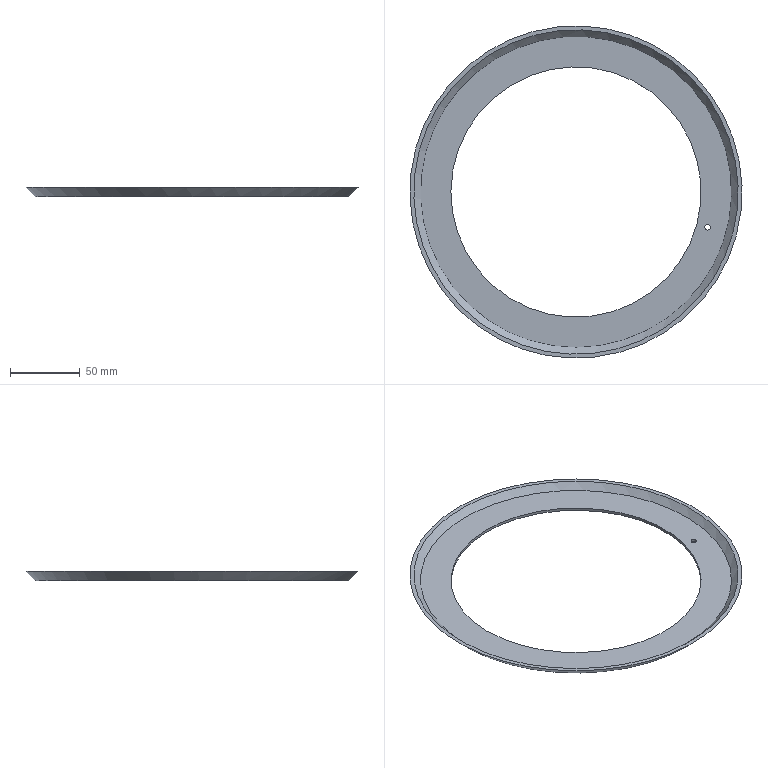Component | NX | OILTHROWRING_2 | 1 solid | 7 faces | box 239 x 239 x 6.75 mm | volume 40152 mm3 | plane 3 | cone 2 | cylinder 2 | commonest cylinder face diameters 4 x1 180 x1
STEP:
#1=CARTESIAN_POINT('',(0.,0.,0.));
#2=DIRECTION('',(0.,0.,1.));
#3=DIRECTION('',(1.,0.,0.));
#4=AXIS2_PLACEMENT_3D('',#1,#2,#3);
#5=CARTESIAN_POINT('',(-108.904,29.181,24.));
#6=VERTEX_POINT('',#5);
#7=CARTESIAN_POINT('',(-0.,0.,24.));
#8=DIRECTION('',(0.,-0.,-1.));
#9=DIRECTION('',(-0.9659,0.2588,-0.));
#10=AXIS2_PLACEMENT_3D('',#7,#8,#9);
#11=CIRCLE('',#10,112.745);
#12=CARTESIAN_POINT('',(108.904,-29.181,24.));
#13=DIRECTION('',(-0.,0.,1.));
#14=DIRECTION('',(0.9659,-0.2588,0.));
#15=AXIS2_PLACEMENT_3D('',#12,#13,#14);
#16=PLANE('',#15);
#17=CARTESIAN_POINT('',(-225.491,0.));
#18=CARTESIAN_POINT('',(-225.491,195.281));
#19=CARTESIAN_POINT('',(-56.373,97.64));
#20=CARTESIAN_POINT('',(112.745,0.));
#21=CARTESIAN_POINT('',(-56.373,-97.64));
#22=CARTESIAN_POINT('',(-225.491,-195.281));
#23=CARTESIAN_POINT('',(-225.491,0.));
#24=(BOUNDED_CURVE()B_SPLINE_CURVE(2,(#17,#18,#19,#20,#21,#22,#23),.UNSPECIFIED.,.T.,.F.)B_SPLINE_CURVE_WITH_KNOTS((1,2,2,2,2,1),(-2.094,0.,2.094,4.189,6.283,8.378),.UNSPECIFIED.)CURVE()GEOMETRIC_REPRESENTATION_ITEM()RATIONAL_B_SPLINE_CURVE((1.,0.5,1.,0.5,1.,0.5,1.))REPRESENTATION_ITEM(''));
#25=(GEOMETRIC_REPRESENTATION_CONTEXT(2)PARAMETRIC_REPRESENTATION_CONTEXT()REPRESENTATION_CONTEXT('',''));
#26=DEFINITIONAL_REPRESENTATION('',(#24),#25);
#27=PCURVE('',#16,#26);
#28=CARTESIAN_POINT('',(-0.,0.,30.755));
#29=DIRECTION('',(-0.,0.,1.));
#30=DIRECTION('',(0.9659,-0.2588,0.));
#31=AXIS2_PLACEMENT_3D('',#28,#29,#30);
#32=CONICAL_SURFACE('',#31,119.5,0.7854);
#33=CARTESIAN_POINT('',(9.425,-6.755));
#34=DIRECTION('',(-1.,0.));
#35=VECTOR('',#34,1.);
#36=LINE('',#33,#35);
#37=(GEOMETRIC_REPRESENTATION_CONTEXT(2)PARAMETRIC_REPRESENTATION_CONTEXT()REPRESENTATION_CONTEXT('',''));
#38=DEFINITIONAL_REPRESENTATION('',(#36),#37);
#39=PCURVE('',#32,#38);
#40=SURFACE_CURVE('',#11,(#27,#39),.PCURVE_S1.);
#41=EDGE_CURVE('',#6,#6,#40,.T.);
#42=ORIENTED_EDGE('',*,*,#41,.T.);
#43=EDGE_LOOP('',(#42));
#44=FACE_BOUND('',#43,.T.);
#45=CARTESIAN_POINT('',(96.593,-25.882,24.));
#46=VERTEX_POINT('',#45);
#47=CARTESIAN_POINT('',(94.661,-25.364,24.));
#48=DIRECTION('',(-0.,0.,1.));
#49=DIRECTION('',(0.9659,-0.2588,0.));
#50=AXIS2_PLACEMENT_3D('',#47,#48,#49);
#51=CIRCLE('',#50,2.);
#52=CARTESIAN_POINT('',(-14.745,0.));
#53=DIRECTION('',(1.,0.));
#54=AXIS2_PLACEMENT_2D('',#52,#53);
#55=CIRCLE('',#54,2.);
#56=(GEOMETRIC_REPRESENTATION_CONTEXT(2)PARAMETRIC_REPRESENTATION_CONTEXT()REPRESENTATION_CONTEXT('',''));
#57=DEFINITIONAL_REPRESENTATION('',(#55),#56);
#58=PCURVE('',#16,#57);
#59=CARTESIAN_POINT('',(94.661,-25.364,24.));
#60=DIRECTION('',(-0.,0.,1.));
#61=DIRECTION('',(0.9659,-0.2588,0.));
#62=AXIS2_PLACEMENT_3D('',#59,#60,#61);
#63=CYLINDRICAL_SURFACE('',#62,2.);
#64=CARTESIAN_POINT('',(0.,0.));
#65=DIRECTION('',(1.,0.));
#66=VECTOR('',#65,1.);
#67=LINE('',#64,#66);
#68=(GEOMETRIC_REPRESENTATION_CONTEXT(2)PARAMETRIC_REPRESENTATION_CONTEXT()REPRESENTATION_CONTEXT('',''));
#69=DEFINITIONAL_REPRESENTATION('',(#67),#68);
#70=PCURVE('',#63,#69);
#71=SURFACE_CURVE('',#51,(#58,#70),.PCURVE_S1.);
#72=EDGE_CURVE('',#46,#46,#71,.T.);
#73=ORIENTED_EDGE('',*,*,#72,.T.);
#74=EDGE_LOOP('',(#73));
#75=FACE_BOUND('',#74,.T.);
#76=CARTESIAN_POINT('',(86.933,-23.294,24.));
#77=VERTEX_POINT('',#76);
#78=CARTESIAN_POINT('',(-0.,0.,24.));
#79=DIRECTION('',(0.,-0.,-1.));
#80=DIRECTION('',(0.9659,-0.2588,0.));
#81=AXIS2_PLACEMENT_3D('',#78,#79,#80);
#82=CIRCLE('',#81,90.);
#83=CARTESIAN_POINT('',(-22.745,0.));
#84=CARTESIAN_POINT('',(-22.745,-155.885));
#85=CARTESIAN_POINT('',(-157.745,-77.942));
#86=CARTESIAN_POINT('',(-292.745,0.));
#87=CARTESIAN_POINT('',(-157.745,77.942));
#88=CARTESIAN_POINT('',(-22.745,155.885));
#89=CARTESIAN_POINT('',(-22.745,0.));
#90=(BOUNDED_CURVE()B_SPLINE_CURVE(2,(#83,#84,#85,#86,#87,#88,#89),.UNSPECIFIED.,.T.,.F.)B_SPLINE_CURVE_WITH_KNOTS((1,2,2,2,2,1),(-2.094,0.,2.094,4.189,6.283,8.378),.UNSPECIFIED.)CURVE()GEOMETRIC_REPRESENTATION_ITEM()RATIONAL_B_SPLINE_CURVE((1.,0.5,1.,0.5,1.,0.5,1.))REPRESENTATION_ITEM(''));
#91=(GEOMETRIC_REPRESENTATION_CONTEXT(2)PARAMETRIC_REPRESENTATION_CONTEXT()REPRESENTATION_CONTEXT('',''));
#92=DEFINITIONAL_REPRESENTATION('',(#90),#91);
#93=PCURVE('',#16,#92);
#94=CARTESIAN_POINT('',(-0.,0.,26.));
#95=DIRECTION('',(0.,-0.,-1.));
#96=DIRECTION('',(-0.9659,0.2588,-0.));
#97=AXIS2_PLACEMENT_3D('',#94,#95,#96);
#98=CYLINDRICAL_SURFACE('',#97,90.);
#99=CARTESIAN_POINT('',(3.142,2.));
#100=DIRECTION('',(1.,0.));
#101=VECTOR('',#100,1.);
#102=LINE('',#99,#101);
#103=(GEOMETRIC_REPRESENTATION_CONTEXT(2)PARAMETRIC_REPRESENTATION_CONTEXT()REPRESENTATION_CONTEXT('',''));
#104=DEFINITIONAL_REPRESENTATION('',(#102),#103);
#105=PCURVE('',#98,#104);
#106=SURFACE_CURVE('',#82,(#93,#105),.PCURVE_S1.);
#107=EDGE_CURVE('',#77,#77,#106,.T.);
#108=ORIENTED_EDGE('',*,*,#107,.F.);
#109=EDGE_LOOP('',(#108));
#110=FACE_BOUND('',#109,.T.);
#111=ADVANCED_FACE('',(#44,#75,#110),#16,.F.);
#112=CARTESIAN_POINT('',(-112.696,30.197,30.755));
#113=VERTEX_POINT('',#112);
#114=CARTESIAN_POINT('',(-0.,0.,30.755));
#115=DIRECTION('',(0.,-0.,-1.));
#116=DIRECTION('',(-0.9659,0.2588,-0.));
#117=AXIS2_PLACEMENT_3D('',#114,#115,#116);
#118=CIRCLE('',#117,116.672);
#119=CARTESIAN_POINT('',(-0.,0.,26.));
#120=DIRECTION('',(-0.,0.,1.));
#121=DIRECTION('',(0.9659,-0.2588,0.));
#122=AXIS2_PLACEMENT_3D('',#119,#120,#121);
#123=CONICAL_SURFACE('',#122,111.917,0.7854);
#124=CARTESIAN_POINT('',(9.425,4.755));
#125=DIRECTION('',(-1.,0.));
#126=VECTOR('',#125,1.);
#127=LINE('',#124,#126);
#128=(GEOMETRIC_REPRESENTATION_CONTEXT(2)PARAMETRIC_REPRESENTATION_CONTEXT()REPRESENTATION_CONTEXT('',''));
#129=DEFINITIONAL_REPRESENTATION('',(#127),#128);
#130=PCURVE('',#123,#129);
#131=CARTESIAN_POINT('',(112.696,-30.197,30.755));
#132=DIRECTION('',(0.,-0.,-1.));
#133=DIRECTION('',(-0.9659,0.2588,-0.));
#134=AXIS2_PLACEMENT_3D('',#131,#132,#133);
#135=PLANE('',#134);
#136=CARTESIAN_POINT('',(116.672,-0.));
#137=DIRECTION('',(1.,0.));
#138=AXIS2_PLACEMENT_2D('',#136,#137);
#139=CIRCLE('',#138,116.672);
#140=(GEOMETRIC_REPRESENTATION_CONTEXT(2)PARAMETRIC_REPRESENTATION_CONTEXT()REPRESENTATION_CONTEXT('',''));
#141=DEFINITIONAL_REPRESENTATION('',(#139),#140);
#142=PCURVE('',#135,#141);
#143=SURFACE_CURVE('',#118,(#130,#142),.PCURVE_S1.);
#144=EDGE_CURVE('',#113,#113,#143,.T.);
#145=ORIENTED_EDGE('',*,*,#144,.T.);
#146=CARTESIAN_POINT('',(-108.103,28.966,26.));
#147=VERTEX_POINT('',#146);
#148=CARTESIAN_POINT('',(-108.103,28.966,26.));
#149=CARTESIAN_POINT('',(-112.696,30.197,30.755));
#150=B_SPLINE_CURVE_WITH_KNOTS('',1,(#148,#149),.UNSPECIFIED.,.F.,.F.,(2,2),(0.,6.724),.PIECEWISE_BEZIER_KNOTS.);
#151=CARTESIAN_POINT('',(3.142,0.));
#152=DIRECTION('',(0.,1.));
#153=VECTOR('',#152,1.);
#154=LINE('',#151,#153);
#155=(GEOMETRIC_REPRESENTATION_CONTEXT(2)PARAMETRIC_REPRESENTATION_CONTEXT()REPRESENTATION_CONTEXT('',''));
#156=DEFINITIONAL_REPRESENTATION('',(#154),#155);
#157=PCURVE('',#123,#156);
#158=CARTESIAN_POINT('',(9.425,0.));
#159=DIRECTION('',(0.,1.));
#160=VECTOR('',#159,1.);
#161=LINE('',#158,#160);
#162=(GEOMETRIC_REPRESENTATION_CONTEXT(2)PARAMETRIC_REPRESENTATION_CONTEXT()REPRESENTATION_CONTEXT('',''));
#163=DEFINITIONAL_REPRESENTATION('',(#161),#162);
#164=PCURVE('',#123,#163);
#165=SEAM_CURVE('',#150,(#157,#164),.PCURVE_S1.);
#166=EDGE_CURVE('',#147,#113,#165,.T.);
#167=ORIENTED_EDGE('',*,*,#166,.F.);
#168=CARTESIAN_POINT('',(-0.,0.,26.));
#169=DIRECTION('',(0.,-0.,-1.));
#170=DIRECTION('',(-0.9659,0.2588,-0.));
#171=AXIS2_PLACEMENT_3D('',#168,#169,#170);
#172=CIRCLE('',#171,111.917);
#173=CARTESIAN_POINT('',(9.425,0.));
#174=DIRECTION('',(-1.,0.));
#175=VECTOR('',#174,1.);
#176=LINE('',#173,#175);
#177=(GEOMETRIC_REPRESENTATION_CONTEXT(2)PARAMETRIC_REPRESENTATION_CONTEXT()REPRESENTATION_CONTEXT('',''));
#178=DEFINITIONAL_REPRESENTATION('',(#176),#177);
#179=PCURVE('',#123,#178);
#180=CARTESIAN_POINT('',(-0.,0.,26.));
#181=DIRECTION('',(0.,-0.,-1.));
#182=DIRECTION('',(-0.9659,0.2588,-0.));
#183=AXIS2_PLACEMENT_3D('',#180,#181,#182);
#184=PLANE('',#183);
#185=CARTESIAN_POINT('',(0.,0.));
#186=DIRECTION('',(1.,0.));
#187=AXIS2_PLACEMENT_2D('',#185,#186);
#188=CIRCLE('',#187,111.917);
#189=(GEOMETRIC_REPRESENTATION_CONTEXT(2)PARAMETRIC_REPRESENTATION_CONTEXT()REPRESENTATION_CONTEXT('',''));
#190=DEFINITIONAL_REPRESENTATION('',(#188),#189);
#191=PCURVE('',#184,#190);
#192=SURFACE_CURVE('',#172,(#179,#191),.PCURVE_S1.);
#193=EDGE_CURVE('',#147,#147,#192,.T.);
#194=ORIENTED_EDGE('',*,*,#193,.F.);
#195=ORIENTED_EDGE('',*,*,#166,.T.);
#196=EDGE_LOOP('',(#145,#167,#194,#195));
#197=FACE_BOUND('',#196,.F.);
#198=ADVANCED_FACE('',(#197),#123,.F.);
#199=CARTESIAN_POINT('',(-115.428,30.929,30.755));
#200=VERTEX_POINT('',#199);
#201=CARTESIAN_POINT('',(-0.,0.,30.755));
#202=DIRECTION('',(0.,-0.,-1.));
#203=DIRECTION('',(-0.9659,0.2588,-0.));
#204=AXIS2_PLACEMENT_3D('',#201,#202,#203);
#205=CIRCLE('',#204,119.5);
#206=CARTESIAN_POINT('',(116.672,-0.));
#207=DIRECTION('',(1.,0.));
#208=AXIS2_PLACEMENT_2D('',#206,#207);
#209=CIRCLE('',#208,119.5);
#210=(GEOMETRIC_REPRESENTATION_CONTEXT(2)PARAMETRIC_REPRESENTATION_CONTEXT()REPRESENTATION_CONTEXT('',''));
#211=DEFINITIONAL_REPRESENTATION('',(#209),#210);
#212=PCURVE('',#135,#211);
#213=CARTESIAN_POINT('',(9.425,0.));
#214=DIRECTION('',(-1.,0.));
#215=VECTOR('',#214,1.);
#216=LINE('',#213,#215);
#217=(GEOMETRIC_REPRESENTATION_CONTEXT(2)PARAMETRIC_REPRESENTATION_CONTEXT()REPRESENTATION_CONTEXT('',''));
#218=DEFINITIONAL_REPRESENTATION('',(#216),#217);
#219=PCURVE('',#32,#218);
#220=SURFACE_CURVE('',#205,(#212,#219),.PCURVE_S1.);
#221=EDGE_CURVE('',#200,#200,#220,.T.);
#222=ORIENTED_EDGE('',*,*,#221,.F.);
#223=EDGE_LOOP('',(#222));
#224=FACE_BOUND('',#223,.T.);
#225=ORIENTED_EDGE('',*,*,#144,.T.);
#226=EDGE_LOOP('',(#225));
#227=FACE_BOUND('',#226,.T.);
#228=ADVANCED_FACE('',(#224,#227),#135,.F.);
#229=ORIENTED_EDGE('',*,*,#41,.F.);
#230=CARTESIAN_POINT('',(-108.904,29.181,24.));
#231=CARTESIAN_POINT('',(-115.428,30.929,30.755));
#232=B_SPLINE_CURVE_WITH_KNOTS('',1,(#230,#231),.UNSPECIFIED.,.F.,.F.,(2,2),(-9.552,0.),.PIECEWISE_BEZIER_KNOTS.);
#233=CARTESIAN_POINT('',(9.425,0.));
#234=DIRECTION('',(0.,1.));
#235=VECTOR('',#234,1.);
#236=LINE('',#233,#235);
#237=(GEOMETRIC_REPRESENTATION_CONTEXT(2)PARAMETRIC_REPRESENTATION_CONTEXT()REPRESENTATION_CONTEXT('',''));
#238=DEFINITIONAL_REPRESENTATION('',(#236),#237);
#239=PCURVE('',#32,#238);
#240=CARTESIAN_POINT('',(3.142,0.));
#241=DIRECTION('',(0.,1.));
#242=VECTOR('',#241,1.);
#243=LINE('',#240,#242);
#244=(GEOMETRIC_REPRESENTATION_CONTEXT(2)PARAMETRIC_REPRESENTATION_CONTEXT()REPRESENTATION_CONTEXT('',''));
#245=DEFINITIONAL_REPRESENTATION('',(#243),#244);
#246=PCURVE('',#32,#245);
#247=SEAM_CURVE('',#232,(#239,#246),.PCURVE_S1.);
#248=EDGE_CURVE('',#6,#200,#247,.T.);
#249=ORIENTED_EDGE('',*,*,#248,.T.);
#250=ORIENTED_EDGE('',*,*,#221,.T.);
#251=ORIENTED_EDGE('',*,*,#248,.F.);
#252=EDGE_LOOP('',(#229,#249,#250,#251));
#253=FACE_BOUND('',#252,.T.);
#254=ADVANCED_FACE('',(#253),#32,.T.);
#255=CARTESIAN_POINT('',(86.933,-23.294,26.));
#256=VERTEX_POINT('',#255);
#257=CARTESIAN_POINT('',(-0.,0.,26.));
#258=DIRECTION('',(0.,-0.,-1.));
#259=DIRECTION('',(0.9659,-0.2588,0.));
#260=AXIS2_PLACEMENT_3D('',#257,#258,#259);
#261=CIRCLE('',#260,90.);
#262=CARTESIAN_POINT('',(-0.,0.));
#263=DIRECTION('',(-1.,-0.));
#264=AXIS2_PLACEMENT_2D('',#262,#263);
#265=CIRCLE('',#264,90.);
#266=(GEOMETRIC_REPRESENTATION_CONTEXT(2)PARAMETRIC_REPRESENTATION_CONTEXT()REPRESENTATION_CONTEXT('',''));
#267=DEFINITIONAL_REPRESENTATION('',(#265),#266);
#268=PCURVE('',#184,#267);
#269=CARTESIAN_POINT('',(3.142,0.));
#270=DIRECTION('',(1.,0.));
#271=VECTOR('',#270,1.);
#272=LINE('',#269,#271);
#273=(GEOMETRIC_REPRESENTATION_CONTEXT(2)PARAMETRIC_REPRESENTATION_CONTEXT()REPRESENTATION_CONTEXT('',''));
#274=DEFINITIONAL_REPRESENTATION('',(#272),#273);
#275=PCURVE('',#98,#274);
#276=SURFACE_CURVE('',#261,(#268,#275),.PCURVE_S1.);
#277=EDGE_CURVE('',#256,#256,#276,.T.);
#278=ORIENTED_EDGE('',*,*,#277,.T.);
#279=EDGE_LOOP('',(#278));
#280=FACE_BOUND('',#279,.T.);
#281=CARTESIAN_POINT('',(92.729,-24.847,26.));
#282=VERTEX_POINT('',#281);
#283=CARTESIAN_POINT('',(96.593,-25.882,26.));
#284=VERTEX_POINT('',#283);
#285=CARTESIAN_POINT('',(94.661,-25.364,26.));
#286=DIRECTION('',(0.,-0.,-1.));
#287=DIRECTION('',(-0.9659,0.2588,-0.));
#288=AXIS2_PLACEMENT_3D('',#285,#286,#287);
#289=CIRCLE('',#288,2.);
#290=CARTESIAN_POINT('',(-98.,-0.));
#291=DIRECTION('',(1.,-0.));
#292=AXIS2_PLACEMENT_2D('',#290,#291);
#293=CIRCLE('',#292,2.);
#294=(GEOMETRIC_REPRESENTATION_CONTEXT(2)PARAMETRIC_REPRESENTATION_CONTEXT()REPRESENTATION_CONTEXT('',''));
#295=DEFINITIONAL_REPRESENTATION('',(#293),#294);
#296=PCURVE('',#184,#295);
#297=CARTESIAN_POINT('',(3.142,2.));
#298=DIRECTION('',(-1.,0.));
#299=VECTOR('',#298,1.);
#300=LINE('',#297,#299);
#301=(GEOMETRIC_REPRESENTATION_CONTEXT(2)PARAMETRIC_REPRESENTATION_CONTEXT()REPRESENTATION_CONTEXT('',''));
#302=DEFINITIONAL_REPRESENTATION('',(#300),#301);
#303=PCURVE('',#63,#302);
#304=SURFACE_CURVE('',#289,(#296,#303),.PCURVE_S1.);
#305=EDGE_CURVE('',#282,#284,#304,.T.);
#306=ORIENTED_EDGE('',*,*,#305,.T.);
#307=CARTESIAN_POINT('',(94.661,-25.364,26.));
#308=DIRECTION('',(0.,-0.,-1.));
#309=DIRECTION('',(-0.9659,0.2588,-0.));
#310=AXIS2_PLACEMENT_3D('',#307,#308,#309);
#311=CIRCLE('',#310,2.);
#312=CARTESIAN_POINT('',(-98.,-0.));
#313=DIRECTION('',(1.,-0.));
#314=AXIS2_PLACEMENT_2D('',#312,#313);
#315=CIRCLE('',#314,2.);
#316=(GEOMETRIC_REPRESENTATION_CONTEXT(2)PARAMETRIC_REPRESENTATION_CONTEXT()REPRESENTATION_CONTEXT('',''));
#317=DEFINITIONAL_REPRESENTATION('',(#315),#316);
#318=PCURVE('',#184,#317);
#319=CARTESIAN_POINT('',(9.425,2.));
#320=DIRECTION('',(-1.,0.));
#321=VECTOR('',#320,1.);
#322=LINE('',#319,#321);
#323=(GEOMETRIC_REPRESENTATION_CONTEXT(2)PARAMETRIC_REPRESENTATION_CONTEXT()REPRESENTATION_CONTEXT('',''));
#324=DEFINITIONAL_REPRESENTATION('',(#322),#323);
#325=PCURVE('',#63,#324);
#326=SURFACE_CURVE('',#311,(#318,#325),.PCURVE_S1.);
#327=EDGE_CURVE('',#284,#282,#326,.T.);
#328=ORIENTED_EDGE('',*,*,#327,.T.);
#329=EDGE_LOOP('',(#306,#328));
#330=FACE_BOUND('',#329,.T.);
#331=ORIENTED_EDGE('',*,*,#193,.F.);
#332=EDGE_LOOP('',(#331));
#333=FACE_BOUND('',#332,.T.);
#334=ADVANCED_FACE('',(#280,#330,#333),#184,.F.);
#335=ORIENTED_EDGE('',*,*,#72,.T.);
#336=CARTESIAN_POINT('',(96.593,-25.882,24.));
#337=CARTESIAN_POINT('',(96.593,-25.882,26.));
#338=B_SPLINE_CURVE_WITH_KNOTS('',1,(#336,#337),.UNSPECIFIED.,.F.,.F.,(2,2),(0.,2.),.PIECEWISE_BEZIER_KNOTS.);
#339=CARTESIAN_POINT('',(6.283,0.));
#340=DIRECTION('',(0.,1.));
#341=VECTOR('',#340,1.);
#342=LINE('',#339,#341);
#343=(GEOMETRIC_REPRESENTATION_CONTEXT(2)PARAMETRIC_REPRESENTATION_CONTEXT()REPRESENTATION_CONTEXT('',''));
#344=DEFINITIONAL_REPRESENTATION('',(#342),#343);
#345=PCURVE('',#63,#344);
#346=CARTESIAN_POINT('',(0.,0.));
#347=DIRECTION('',(0.,1.));
#348=VECTOR('',#347,1.);
#349=LINE('',#346,#348);
#350=(GEOMETRIC_REPRESENTATION_CONTEXT(2)PARAMETRIC_REPRESENTATION_CONTEXT()REPRESENTATION_CONTEXT('',''));
#351=DEFINITIONAL_REPRESENTATION('',(#349),#350);
#352=PCURVE('',#63,#351);
#353=SEAM_CURVE('',#338,(#345,#352),.PCURVE_S1.);
#354=EDGE_CURVE('',#46,#284,#353,.T.);
#355=ORIENTED_EDGE('',*,*,#354,.T.);
#356=ORIENTED_EDGE('',*,*,#327,.T.);
#357=ORIENTED_EDGE('',*,*,#305,.T.);
#358=ORIENTED_EDGE('',*,*,#354,.F.);
#359=EDGE_LOOP('',(#335,#355,#356,#357,#358));
#360=FACE_BOUND('',#359,.F.);
#361=ADVANCED_FACE('',(#360),#63,.F.);
#362=ORIENTED_EDGE('',*,*,#277,.T.);
#363=CARTESIAN_POINT('',(86.933,-23.294,26.));
#364=CARTESIAN_POINT('',(86.933,-23.294,24.));
#365=B_SPLINE_CURVE_WITH_KNOTS('',1,(#363,#364),.UNSPECIFIED.,.F.,.F.,(2,2),(0.,2.),.PIECEWISE_BEZIER_KNOTS.);
#366=CARTESIAN_POINT('',(9.425,0.));
#367=DIRECTION('',(0.,1.));
#368=VECTOR('',#367,1.);
#369=LINE('',#366,#368);
#370=(GEOMETRIC_REPRESENTATION_CONTEXT(2)PARAMETRIC_REPRESENTATION_CONTEXT()REPRESENTATION_CONTEXT('',''));
#371=DEFINITIONAL_REPRESENTATION('',(#369),#370);
#372=PCURVE('',#98,#371);
#373=CARTESIAN_POINT('',(3.142,0.));
#374=DIRECTION('',(0.,1.));
#375=VECTOR('',#374,1.);
#376=LINE('',#373,#375);
#377=(GEOMETRIC_REPRESENTATION_CONTEXT(2)PARAMETRIC_REPRESENTATION_CONTEXT()REPRESENTATION_CONTEXT('',''));
#378=DEFINITIONAL_REPRESENTATION('',(#376),#377);
#379=PCURVE('',#98,#378);
#380=SEAM_CURVE('',#365,(#372,#379),.PCURVE_S1.);
#381=EDGE_CURVE('',#256,#77,#380,.T.);
#382=ORIENTED_EDGE('',*,*,#381,.T.);
#383=ORIENTED_EDGE('',*,*,#107,.F.);
#384=ORIENTED_EDGE('',*,*,#381,.F.);
#385=EDGE_LOOP('',(#362,#382,#383,#384));
#386=FACE_BOUND('',#385,.F.);
#387=ADVANCED_FACE('',(#386),#98,.F.);
#388=CLOSED_SHELL('',(#111,#198,#228,#254,#334,#361,#387));
#389=MANIFOLD_SOLID_BREP('',#388);
#390=(LENGTH_UNIT()NAMED_UNIT(*)SI_UNIT(.MILLI.,.METRE.));
#391=UNCERTAINTY_MEASURE_WITH_UNIT(LENGTH_MEASURE(0.000005),#390,'','');
#392=(NAMED_UNIT(*)PLANE_ANGLE_UNIT()SI_UNIT($,.RADIAN.));
#393=(NAMED_UNIT(*)SI_UNIT($,.STERADIAN.)SOLID_ANGLE_UNIT());
#394=(GEOMETRIC_REPRESENTATION_CONTEXT(3)GLOBAL_UNCERTAINTY_ASSIGNED_CONTEXT((#391))GLOBAL_UNIT_ASSIGNED_CONTEXT((#390,#392,#393))REPRESENTATION_CONTEXT('',''));
#395=ADVANCED_BREP_SHAPE_REPRESENTATION('',(#4,#389),#394);